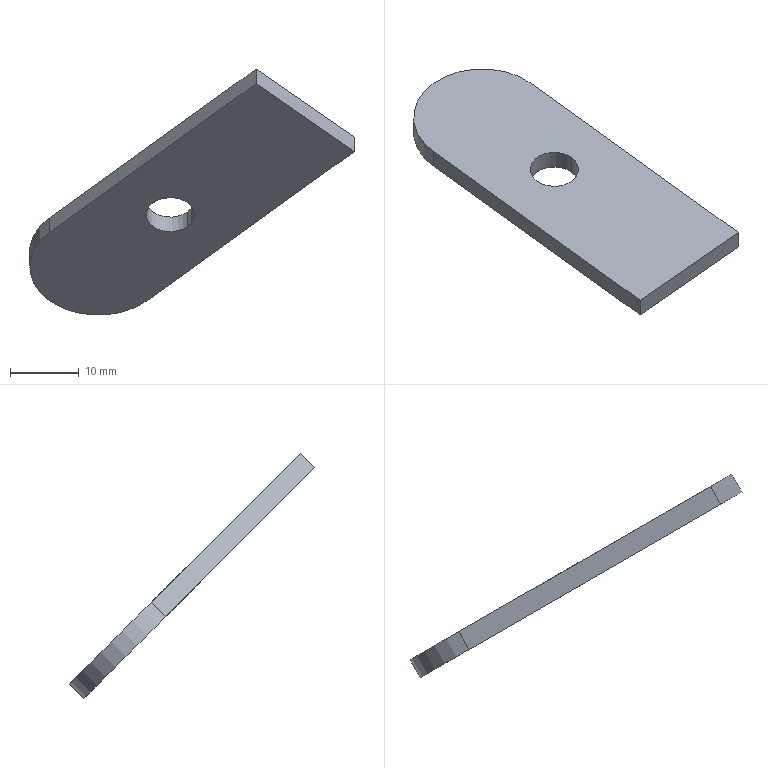Component | SolidWorks | SmallAxisAssembly-1_AdjustingWheelEar-1 | 1 solid | 8 faces | box 47.26 x 35.85 x 35.84 mm | volume 2936 mm3 | plane 5 | cylinder 3 | commonest cylinder face diameters 7 x2 20 x1
build123d program:
from build123d import *

# Parameters (mm, degrees)
SKETCH1_R           = 3.5
BOSS_EXTRUDE1_DEPTH = 3


with BuildPart() as part:
    # Sketch1 → Boss-Extrude1 (new body)
    with BuildSketch(Plane.XY):
        with BuildLine():
            Line((10, 0), (-10, 0))
            Line((-10, 0), (-10, 43))
            ThreePointArc((-10, 43), (0, 53), (10, 43))
            Line((10, 43), (10, 0))
        make_face()
        with Locations((0, 28)):
            Circle(SKETCH1_R, mode=Mode.SUBTRACT)
    extrude(amount=BOSS_EXTRUDE1_DEPTH)


solid = part.part

# Placed as in the assembly
solid = solid.moved(Location((-22.105, 852.728, 285.537), (-45, 0.02994, 44.465)))
STEP:
#1=COLOUR_RGB('',0.7922,0.8196,0.9333);
#2=FILL_AREA_STYLE_COLOUR('',#1);
#3=FILL_AREA_STYLE('',(#2));
#4=SURFACE_STYLE_FILL_AREA(#3);
#5=SURFACE_SIDE_STYLE('',(#4));
#6=SURFACE_STYLE_USAGE(.BOTH.,#5);
#7=PRESENTATION_STYLE_ASSIGNMENT((#6));
#8=CARTESIAN_POINT('',(-1.544,34.197,10.617));
#9=VERTEX_POINT('',#8);
#10=CARTESIAN_POINT('',(-1.741,34.06,10.754));
#11=VERTEX_POINT('',#10);
#12=CARTESIAN_POINT('',(-1.642,34.129,10.686));
#13=DIRECTION('',(-0.0005225,-0.7071,-0.7071));
#14=DIRECTION('',(-0.7137,-0.495,0.4956));
#15=AXIS2_PLACEMENT_3D('',#12,#13,#14);
#16=CIRCLE('',#15,0.1378);
#17=EDGE_CURVE('',#9,#11,#16,.T.);
#18=ORIENTED_EDGE('',*,*,#17,.T.);
#19=CARTESIAN_POINT('',(-1.741,34.144,10.837));
#20=VERTEX_POINT('',#19);
#21=CARTESIAN_POINT('',(-1.741,34.06,10.754));
#22=DIRECTION('',(0.0005225,0.7071,0.7071));
#23=VECTOR('',#22,39.37);
#24=LINE('',#21,#23);
#25=EDGE_CURVE('',#11,#20,#24,.T.);
#26=ORIENTED_EDGE('',*,*,#25,.T.);
#27=CARTESIAN_POINT('',(-1.544,34.28,10.701));
#28=VERTEX_POINT('',#27);
#29=CARTESIAN_POINT('',(-1.642,34.212,10.769));
#30=DIRECTION('',(-0.0005225,-0.7071,-0.7071));
#31=DIRECTION('',(-0.7137,-0.495,0.4956));
#32=AXIS2_PLACEMENT_3D('',#29,#30,#31);
#33=CIRCLE('',#32,0.1378);
#34=EDGE_CURVE('',#28,#20,#33,.T.);
#35=ORIENTED_EDGE('',*,*,#34,.F.);
#36=CARTESIAN_POINT('',(-1.544,34.197,10.617));
#37=DIRECTION('',(0.0005225,0.7071,0.7071));
#38=VECTOR('',#37,39.37);
#39=LINE('',#36,#38);
#40=EDGE_CURVE('',#9,#28,#39,.T.);
#41=ORIENTED_EDGE('',*,*,#40,.F.);
#42=EDGE_LOOP('',(#18,#26,#35,#41));
#43=FACE_OUTER_BOUND('',#42,.T.);
#44=CARTESIAN_POINT('',(-1.642,34.129,10.686));
#45=DIRECTION('',(0.0005225,0.7071,0.7071));
#46=DIRECTION('',(0.7137,0.495,-0.4956));
#47=AXIS2_PLACEMENT_3D('',#44,#45,#46);
#48=CYLINDRICAL_SURFACE('',#47,0.1378);
#49=ADVANCED_FACE('',(#43),#48,.F.);
#50=CARTESIAN_POINT('',(-1.775,34.622,10.193));
#51=VERTEX_POINT('',#50);
#52=CARTESIAN_POINT('',(-0.5893,33.767,11.046));
#53=VERTEX_POINT('',#52);
#54=CARTESIAN_POINT('',(-0.5893,33.767,11.046));
#55=DIRECTION('',(0.7005,-0.5049,0.5044));
#56=VECTOR('',#55,39.37);
#57=LINE('',#54,#56);
#58=EDGE_CURVE('',#51,#53,#57,.T.);
#59=ORIENTED_EDGE('',*,*,#58,.T.);
#60=CARTESIAN_POINT('',(-1.151,33.377,11.437));
#61=VERTEX_POINT('',#60);
#62=CARTESIAN_POINT('',(-1.151,33.377,11.437));
#63=DIRECTION('',(-0.7137,-0.495,0.4956));
#64=VECTOR('',#63,39.37);
#65=LINE('',#62,#64);
#66=EDGE_CURVE('',#53,#61,#65,.T.);
#67=ORIENTED_EDGE('',*,*,#66,.T.);
#68=CARTESIAN_POINT('',(-2.337,34.232,10.583));
#69=VERTEX_POINT('',#68);
#70=CARTESIAN_POINT('',(-2.337,34.232,10.583));
#71=DIRECTION('',(-0.7005,0.5049,-0.5044));
#72=VECTOR('',#71,39.37);
#73=LINE('',#70,#72);
#74=EDGE_CURVE('',#61,#69,#73,.T.);
#75=ORIENTED_EDGE('',*,*,#74,.T.);
#76=CARTESIAN_POINT('',(-2.056,34.427,10.388));
#77=DIRECTION('',(-0.0005225,-0.7071,-0.7071));
#78=DIRECTION('',(0.7137,0.495,-0.4956));
#79=AXIS2_PLACEMENT_3D('',#76,#77,#78);
#80=CIRCLE('',#79,0.3937);
#81=EDGE_CURVE('',#69,#51,#80,.T.);
#82=ORIENTED_EDGE('',*,*,#81,.T.);
#83=EDGE_LOOP('',(#59,#67,#75,#82));
#84=FACE_OUTER_BOUND('',#83,.T.);
#85=ORIENTED_EDGE('',*,*,#17,.F.);
#86=CARTESIAN_POINT('',(-1.642,34.129,10.686));
#87=DIRECTION('',(-0.0005225,-0.7071,-0.7071));
#88=DIRECTION('',(-0.7137,-0.495,0.4956));
#89=AXIS2_PLACEMENT_3D('',#86,#87,#88);
#90=CIRCLE('',#89,0.1378);
#91=EDGE_CURVE('',#11,#9,#90,.T.);
#92=ORIENTED_EDGE('',*,*,#91,.F.);
#93=EDGE_LOOP('',(#85,#92));
#94=FACE_BOUND('',#93,.T.);
#95=CARTESIAN_POINT('',(-2.056,34.427,10.388));
#96=DIRECTION('',(0.0005225,0.7071,0.7071));
#97=DIRECTION('',(0.7137,0.495,-0.4956));
#98=AXIS2_PLACEMENT_3D('',#95,#96,#97);
#99=PLANE('',#98);
#100=ADVANCED_FACE('',(#84,#94),#99,.F.);
#101=CARTESIAN_POINT('',(-1.775,34.705,10.276));
#102=VERTEX_POINT('',#101);
#103=CARTESIAN_POINT('',(-0.5892,33.85,11.13));
#104=VERTEX_POINT('',#103);
#105=CARTESIAN_POINT('',(-0.5892,33.85,11.13));
#106=DIRECTION('',(0.7005,-0.5049,0.5044));
#107=VECTOR('',#106,39.37);
#108=LINE('',#105,#107);
#109=EDGE_CURVE('',#102,#104,#108,.T.);
#110=ORIENTED_EDGE('',*,*,#109,.F.);
#111=CARTESIAN_POINT('',(-2.337,34.315,10.666));
#112=VERTEX_POINT('',#111);
#113=CARTESIAN_POINT('',(-2.056,34.51,10.471));
#114=DIRECTION('',(-0.0005225,-0.7071,-0.7071));
#115=DIRECTION('',(0.7137,0.495,-0.4956));
#116=AXIS2_PLACEMENT_3D('',#113,#114,#115);
#117=CIRCLE('',#116,0.3937);
#118=EDGE_CURVE('',#112,#102,#117,.T.);
#119=ORIENTED_EDGE('',*,*,#118,.F.);
#120=CARTESIAN_POINT('',(-1.151,33.461,11.52));
#121=VERTEX_POINT('',#120);
#122=CARTESIAN_POINT('',(-2.337,34.315,10.666));
#123=DIRECTION('',(-0.7005,0.5049,-0.5044));
#124=VECTOR('',#123,39.37);
#125=LINE('',#122,#124);
#126=EDGE_CURVE('',#121,#112,#125,.T.);
#127=ORIENTED_EDGE('',*,*,#126,.F.);
#128=CARTESIAN_POINT('',(-1.151,33.461,11.52));
#129=DIRECTION('',(-0.7137,-0.495,0.4956));
#130=VECTOR('',#129,39.37);
#131=LINE('',#128,#130);
#132=EDGE_CURVE('',#104,#121,#131,.T.);
#133=ORIENTED_EDGE('',*,*,#132,.F.);
#134=EDGE_LOOP('',(#110,#119,#127,#133));
#135=FACE_OUTER_BOUND('',#134,.T.);
#136=ORIENTED_EDGE('',*,*,#34,.T.);
#137=CARTESIAN_POINT('',(-1.642,34.212,10.769));
#138=DIRECTION('',(-0.0005225,-0.7071,-0.7071));
#139=DIRECTION('',(-0.7137,-0.495,0.4956));
#140=AXIS2_PLACEMENT_3D('',#137,#138,#139);
#141=CIRCLE('',#140,0.1378);
#142=EDGE_CURVE('',#20,#28,#141,.T.);
#143=ORIENTED_EDGE('',*,*,#142,.T.);
#144=EDGE_LOOP('',(#136,#143));
#145=FACE_BOUND('',#144,.T.);
#146=CARTESIAN_POINT('',(-2.056,34.51,10.471));
#147=DIRECTION('',(0.0005225,0.7071,0.7071));
#148=DIRECTION('',(0.7137,0.495,-0.4956));
#149=AXIS2_PLACEMENT_3D('',#146,#147,#148);
#150=PLANE('',#149);
#151=ADVANCED_FACE('',(#135,#145),#150,.T.);
#152=ORIENTED_EDGE('',*,*,#109,.T.);
#153=CARTESIAN_POINT('',(-0.5893,33.767,11.046));
#154=DIRECTION('',(0.0005225,0.7071,0.7071));
#155=VECTOR('',#154,39.37);
#156=LINE('',#153,#155);
#157=EDGE_CURVE('',#53,#104,#156,.T.);
#158=ORIENTED_EDGE('',*,*,#157,.F.);
#159=ORIENTED_EDGE('',*,*,#58,.F.);
#160=CARTESIAN_POINT('',(-1.775,34.622,10.193));
#161=DIRECTION('',(0.0005225,0.7071,0.7071));
#162=VECTOR('',#161,39.37);
#163=LINE('',#160,#162);
#164=EDGE_CURVE('',#51,#102,#163,.T.);
#165=ORIENTED_EDGE('',*,*,#164,.T.);
#166=EDGE_LOOP('',(#152,#158,#159,#165));
#167=FACE_OUTER_BOUND('',#166,.T.);
#168=CARTESIAN_POINT('',(-0.5893,33.767,11.046));
#169=DIRECTION('',(-0.7137,-0.495,0.4956));
#170=DIRECTION('',(-0.7005,0.5049,-0.5044));
#171=AXIS2_PLACEMENT_3D('',#168,#169,#170);
#172=PLANE('',#171);
#173=ADVANCED_FACE('',(#167),#172,.F.);
#174=ORIENTED_EDGE('',*,*,#132,.T.);
#175=CARTESIAN_POINT('',(-1.151,33.377,11.437));
#176=DIRECTION('',(0.0005225,0.7071,0.7071));
#177=VECTOR('',#176,39.37);
#178=LINE('',#175,#177);
#179=EDGE_CURVE('',#61,#121,#178,.T.);
#180=ORIENTED_EDGE('',*,*,#179,.F.);
#181=ORIENTED_EDGE('',*,*,#66,.F.);
#182=ORIENTED_EDGE('',*,*,#157,.T.);
#183=EDGE_LOOP('',(#174,#180,#181,#182));
#184=FACE_OUTER_BOUND('',#183,.T.);
#185=CARTESIAN_POINT('',(-1.151,33.377,11.437));
#186=DIRECTION('',(-0.7005,0.5049,-0.5044));
#187=DIRECTION('',(0.7137,0.495,-0.4956));
#188=AXIS2_PLACEMENT_3D('',#185,#186,#187);
#189=PLANE('',#188);
#190=ADVANCED_FACE('',(#184),#189,.F.);
#191=ORIENTED_EDGE('',*,*,#126,.T.);
#192=CARTESIAN_POINT('',(-2.337,34.232,10.583));
#193=DIRECTION('',(0.0005225,0.7071,0.7071));
#194=VECTOR('',#193,39.37);
#195=LINE('',#192,#194);
#196=EDGE_CURVE('',#69,#112,#195,.T.);
#197=ORIENTED_EDGE('',*,*,#196,.F.);
#198=ORIENTED_EDGE('',*,*,#74,.F.);
#199=ORIENTED_EDGE('',*,*,#179,.T.);
#200=EDGE_LOOP('',(#191,#197,#198,#199));
#201=FACE_OUTER_BOUND('',#200,.T.);
#202=CARTESIAN_POINT('',(-2.337,34.232,10.583));
#203=DIRECTION('',(0.7137,0.495,-0.4956));
#204=DIRECTION('',(0.7005,-0.5049,0.5044));
#205=AXIS2_PLACEMENT_3D('',#202,#203,#204);
#206=PLANE('',#205);
#207=ADVANCED_FACE('',(#201),#206,.F.);
#208=ORIENTED_EDGE('',*,*,#118,.T.);
#209=ORIENTED_EDGE('',*,*,#164,.F.);
#210=ORIENTED_EDGE('',*,*,#81,.F.);
#211=ORIENTED_EDGE('',*,*,#196,.T.);
#212=EDGE_LOOP('',(#208,#209,#210,#211));
#213=FACE_OUTER_BOUND('',#212,.T.);
#214=CARTESIAN_POINT('',(-2.056,34.427,10.388));
#215=DIRECTION('',(0.0005225,0.7071,0.7071));
#216=DIRECTION('',(0.7137,0.495,-0.4956));
#217=AXIS2_PLACEMENT_3D('',#214,#215,#216);
#218=CYLINDRICAL_SURFACE('',#217,0.3937);
#219=ADVANCED_FACE('',(#213),#218,.T.);
#220=ORIENTED_EDGE('',*,*,#25,.F.);
#221=ORIENTED_EDGE('',*,*,#91,.T.);
#222=ORIENTED_EDGE('',*,*,#40,.T.);
#223=ORIENTED_EDGE('',*,*,#142,.F.);
#224=EDGE_LOOP('',(#220,#221,#222,#223));
#225=FACE_OUTER_BOUND('',#224,.T.);
#226=CARTESIAN_POINT('',(-1.642,34.129,10.686));
#227=DIRECTION('',(0.0005225,0.7071,0.7071));
#228=DIRECTION('',(0.7137,0.495,-0.4956));
#229=AXIS2_PLACEMENT_3D('',#226,#227,#228);
#230=CYLINDRICAL_SURFACE('',#229,0.1378);
#231=ADVANCED_FACE('',(#225),#230,.F.);
#232=CLOSED_SHELL('',(#49,#100,#151,#173,#190,#207,#219,#231));
#233=MANIFOLD_SOLID_BREP('',#232);
#234=STYLED_ITEM('',(#7),#233);
#235=PRESENTATION_LAYER_ASSIGNMENT('','',(#234));
#236=(LENGTH_UNIT()NAMED_UNIT(*)SI_UNIT($,.METRE.));
#237=LENGTH_MEASURE_WITH_UNIT(LENGTH_MEASURE(0.0254),#236);
#238=DIMENSIONAL_EXPONENTS(1.,0.,0.,0.,0.,0.,0.);
#239=(CONVERSION_BASED_UNIT('',#237)LENGTH_UNIT()NAMED_UNIT(#238));
#240=UNCERTAINTY_MEASURE_WITH_UNIT(LENGTH_MEASURE(0.00001),#239,'','');
#241=(NAMED_UNIT(*)PLANE_ANGLE_UNIT()SI_UNIT($,.RADIAN.));
#242=(NAMED_UNIT(*)SI_UNIT($,.STERADIAN.)SOLID_ANGLE_UNIT());
#243=(GEOMETRIC_REPRESENTATION_CONTEXT(3)GLOBAL_UNCERTAINTY_ASSIGNED_CONTEXT((#240))GLOBAL_UNIT_ASSIGNED_CONTEXT((#239,#241,#242))REPRESENTATION_CONTEXT('',''));
#244=MECHANICAL_DESIGN_GEOMETRIC_PRESENTATION_REPRESENTATION('',(#234),#243);
#245=CARTESIAN_POINT('',(0.,0.,0.));
#246=DIRECTION('',(0.,0.,1.));
#247=DIRECTION('',(1.,0.,0.));
#248=AXIS2_PLACEMENT_3D('',#245,#246,#247);
#249=(LENGTH_UNIT()NAMED_UNIT(*)SI_UNIT($,.METRE.));
#250=LENGTH_MEASURE_WITH_UNIT(LENGTH_MEASURE(0.0254),#249);
#251=DIMENSIONAL_EXPONENTS(1.,0.,0.,0.,0.,0.,0.);
#252=(CONVERSION_BASED_UNIT('',#250)LENGTH_UNIT()NAMED_UNIT(#251));
#253=UNCERTAINTY_MEASURE_WITH_UNIT(LENGTH_MEASURE(0.00001),#252,'','');
#254=(NAMED_UNIT(*)PLANE_ANGLE_UNIT()SI_UNIT($,.RADIAN.));
#255=(NAMED_UNIT(*)SI_UNIT($,.STERADIAN.)SOLID_ANGLE_UNIT());
#256=(GEOMETRIC_REPRESENTATION_CONTEXT(3)GLOBAL_UNCERTAINTY_ASSIGNED_CONTEXT((#253))GLOBAL_UNIT_ASSIGNED_CONTEXT((#252,#254,#255))REPRESENTATION_CONTEXT('',''));
#257=ADVANCED_BREP_SHAPE_REPRESENTATION('',(#233,#248),#256);